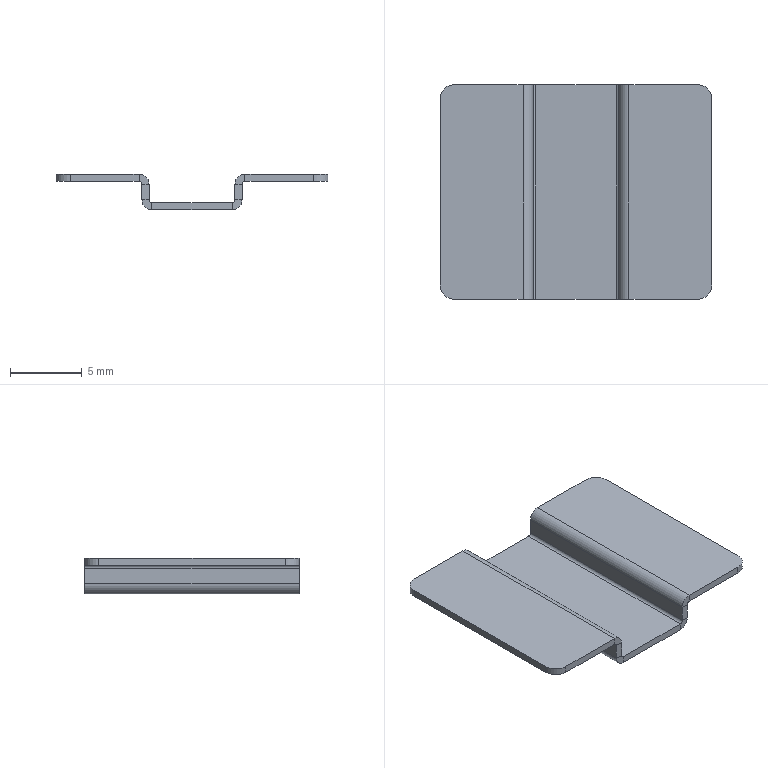Component | SolidWorks | 2018SOLIDWORKS1400000501-1 | 1 solid | 42 faces | box 19 x 15 x 2.5 mm | volume 166 mm3 | plane 30 | cylinder 12 | commonest cylinder face diameters 1.4 x4 0.4 x4 2 x4 | material SUS 304